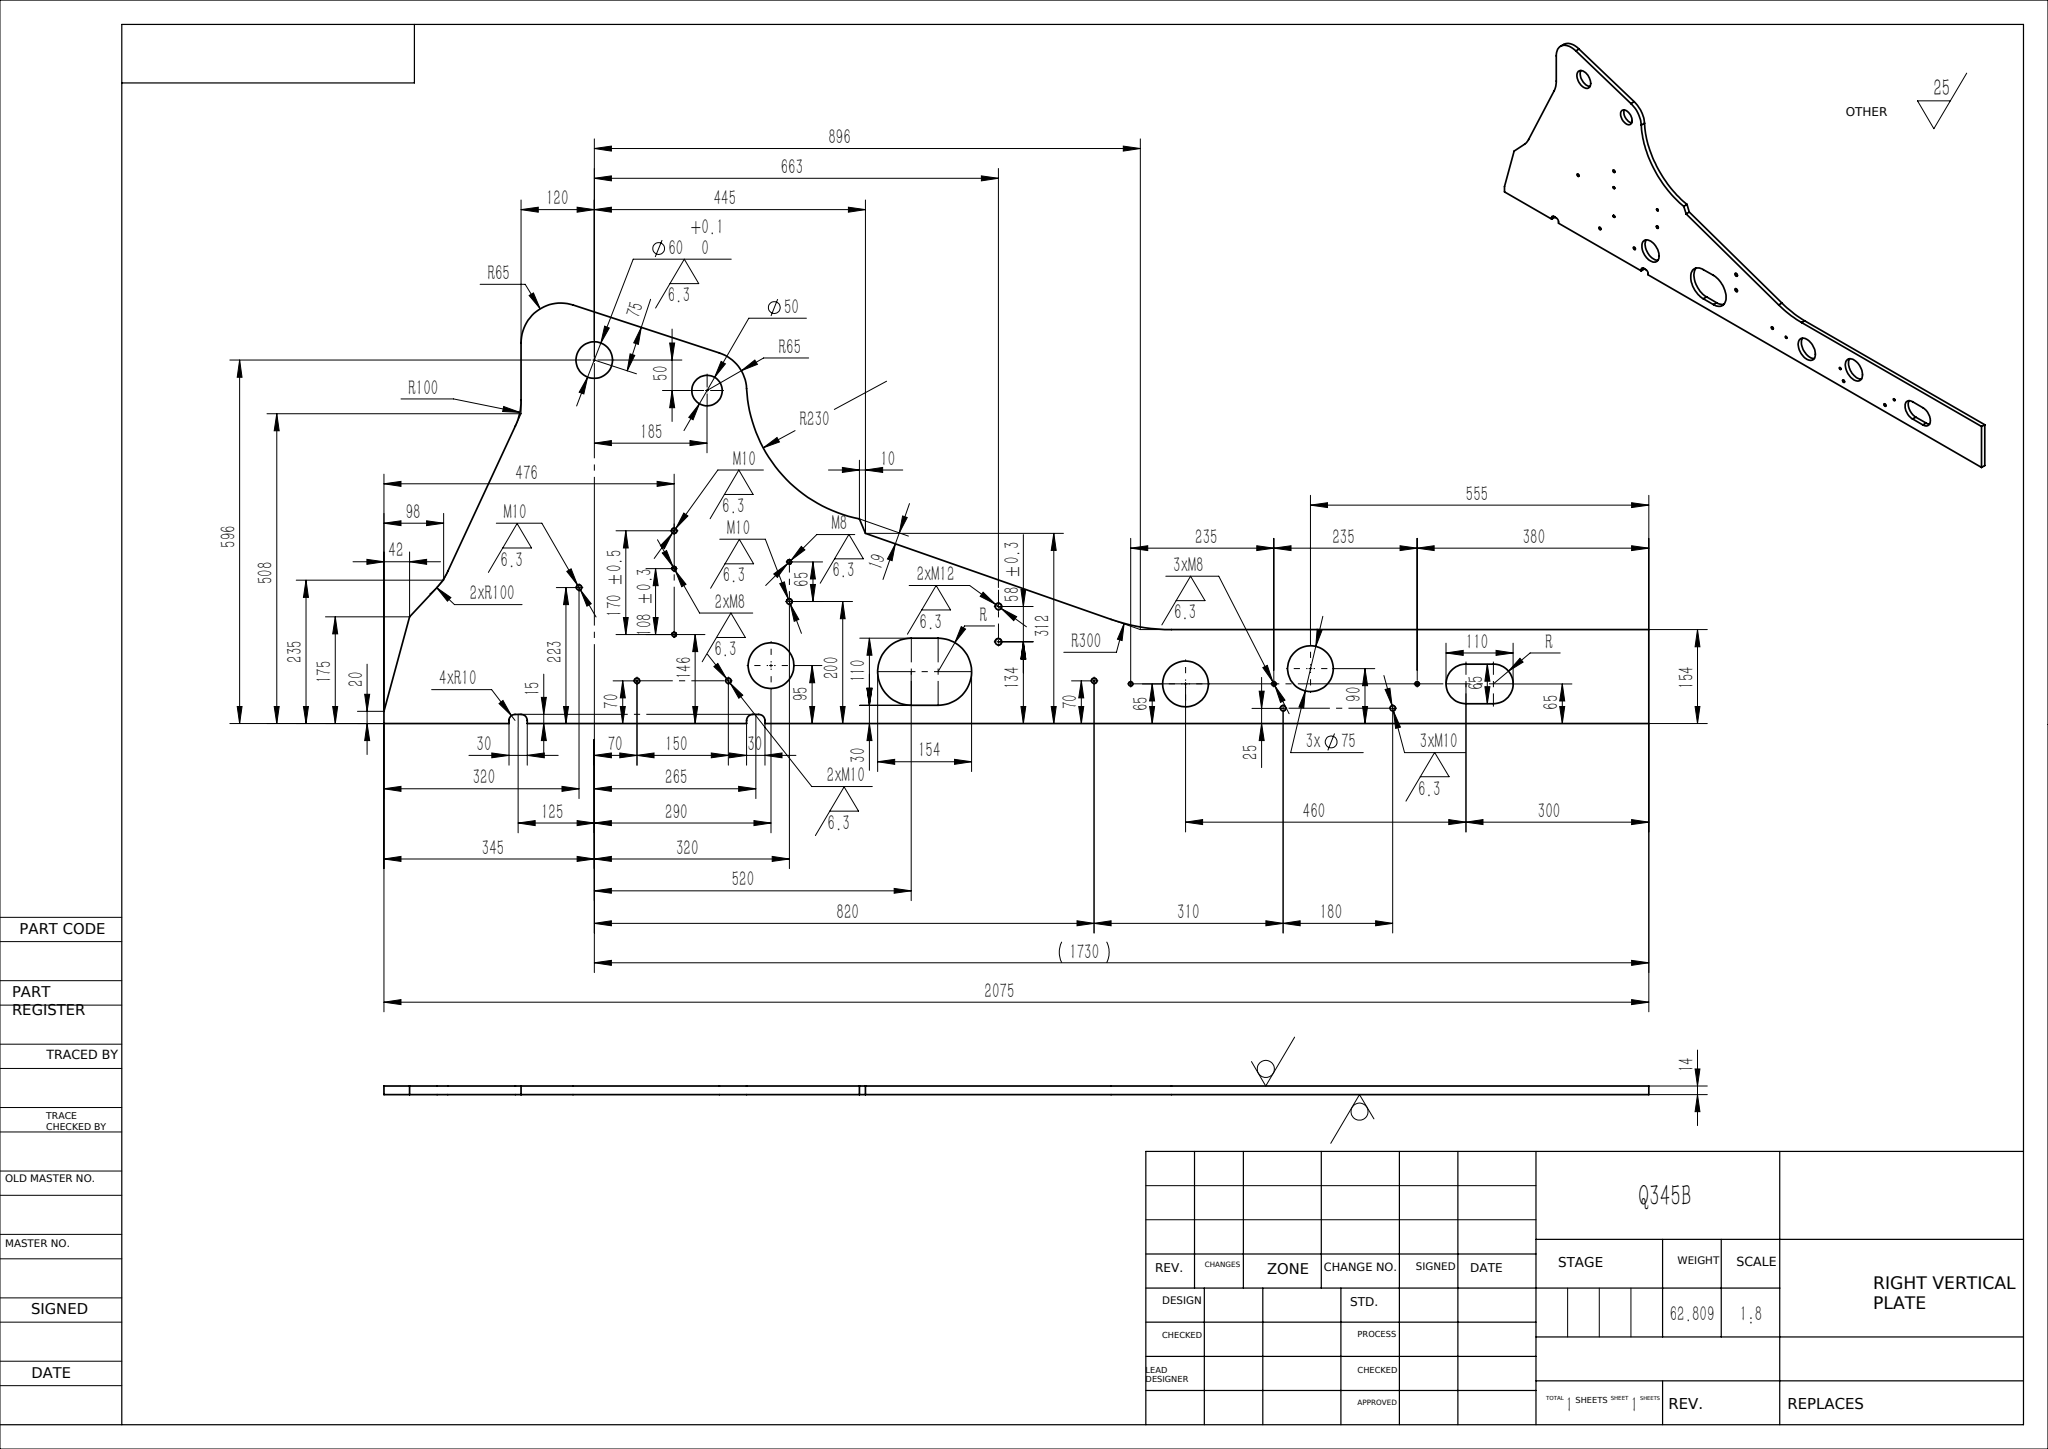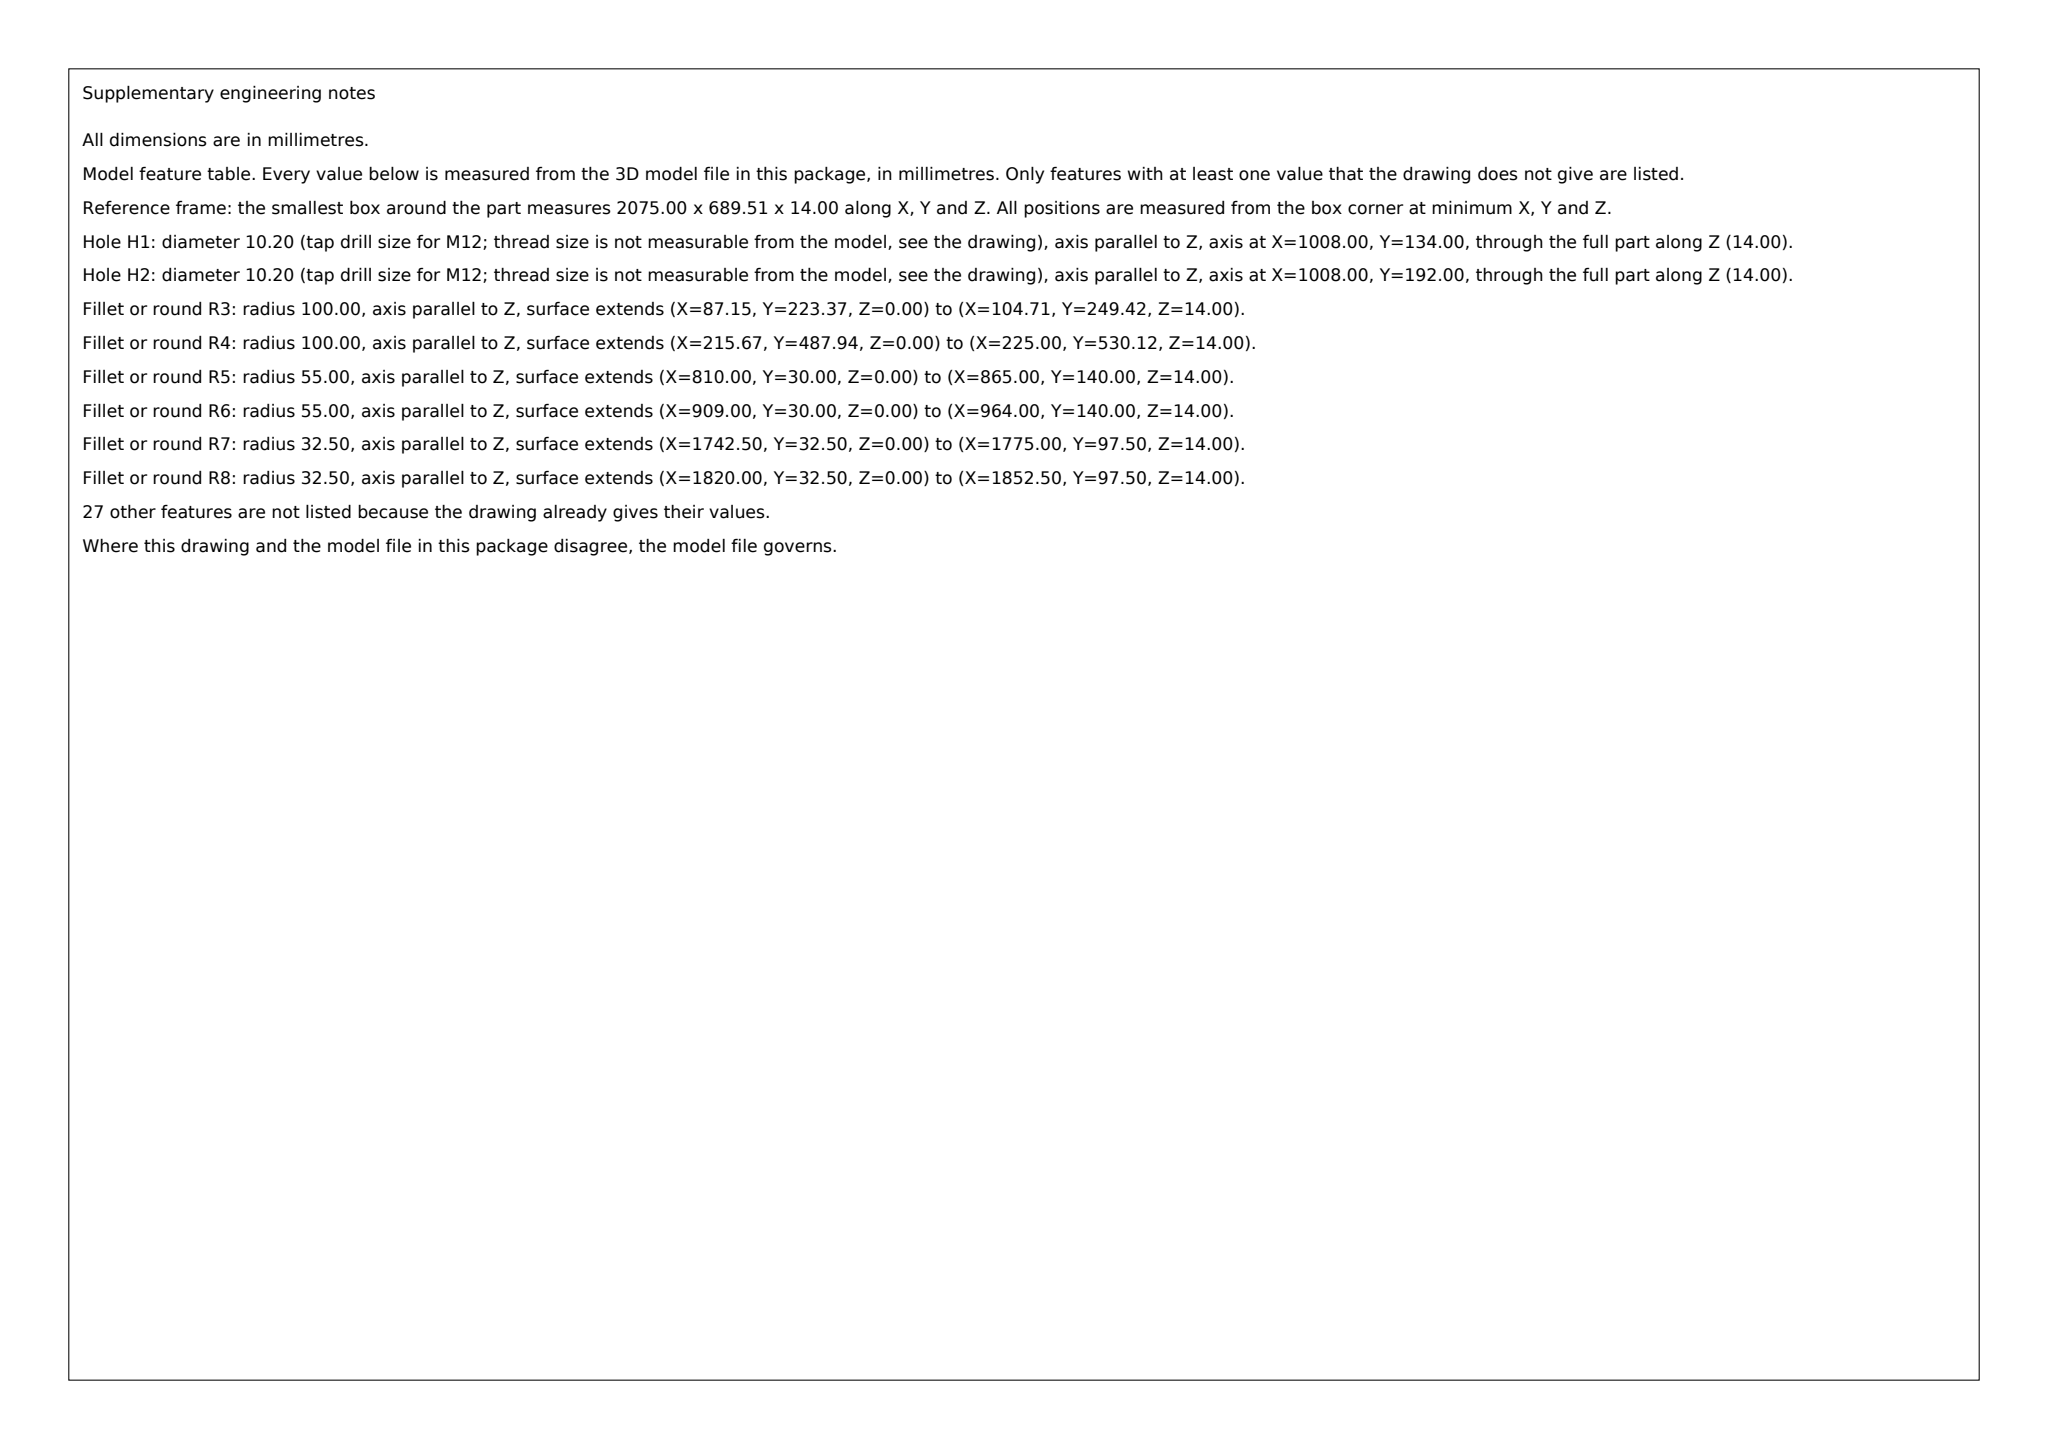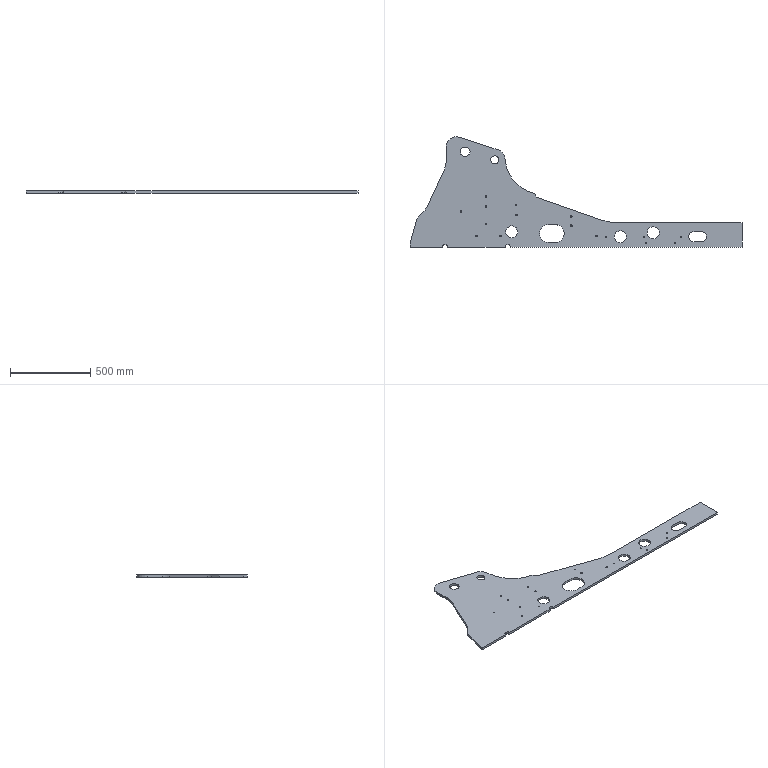Part | SolidWorks | mm | material Q345B | 1 solid | 83 faces | box 2075 x 689.51 x 14 mm | volume 8001084 mm3 | cylinder 58 | plane 25 | commonest cylinder face diameters 8.5 x16 6.8 x12 75 x6 10.2 x4 20 x4 110 x3 65 x3 50 x2
build123d program:
from build123d import *

# Parameters (mm, degrees)
SKETCH1_R           = 30
SKETCH1_R_2         = 37.5
SKETCH1_R_3         = 25
BOSS_EXTRUDE1_DEPTH = 14
M10_TAPPED_HOLE1_D  = 8.5
M10_TAPPED_HOLE2_D  = 8.5
M8_TAPPED_HOLE1_D   = 6.8
M10_TAPPED_HOLE4_D  = 8.5
M8_TAPPED_HOLE3_D   = 6.8
M12_TAPPED_HOLE1_D  = 10.2
M10_TAPPED_HOLE3_D  = 8.5
M8_TAPPED_HOLE4_D   = 6.8


with BuildPart() as part:
    # Sketch1 → Boss-Extrude1 (new body)
    with BuildSketch(Plane.XY):
        with BuildLine():
            Line((0, 0), (205, 0))
            Line((205, 0), (205, 5))
            ThreePointArc((205, 5), (207.929, 12.071), (215, 15))
            Line((215, 15), (225, 15))
            ThreePointArc((225, 15), (232.071, 12.071), (235, 5))
            Line((235, 5), (235, 0))
            Line((235, 0), (595, 0))
            Line((595, 0), (595, 5))
            ThreePointArc((595, 5), (597.929, 12.071), (605, 15))
            Line((605, 15), (615, 15))
            ThreePointArc((615, 15), (622.071, 12.071), (625, 5))
            Line((625, 5), (625, 0))
            Line((625, 0), (2075, 0))
            Line((2075, 0), (2075, 154))
            Line((2075, 154), (1292.029, 154))
            ThreePointArc((1292.029, 154), (1241.723, 158.248), (1192.84, 170.872))
            Line((1192.84, 170.872), (790, 312))
            Line((790, 312), (780, 335.636))
            ThreePointArc((780, 335.636), (650.738, 410.702), (594.913, 549.364))
            ThreePointArc((594.913, 549.364), (581.619, 585.503), (550.21, 607.778))
            Line((550.21, 607.778), (310.21, 686.293))
            ThreePointArc((310.21, 686.293), (251.847, 677.139), (225, 624.514))
            Line((225, 624.514), (225, 530.122))
            ThreePointArc((225, 530.122), (222.639, 508.522), (215.669, 487.942))
            Line((215.669, 487.942), (104.71, 249.423))
            ThreePointArc((104.71, 249.423), (96.957, 235.703), (87.146, 223.371))
            Line((87.146, 223.371), (42, 175))
            Line((42, 175), (0, 20))
            Line((0, 20), (0, 0))
        make_face()
        with Locations((345, 596)):
            Circle(SKETCH1_R, mode=Mode.SUBTRACT)
        with Locations((1520, 90)):
            Circle(SKETCH1_R_2, mode=Mode.SUBTRACT)
        with Locations((1315, 65)):
            Circle(SKETCH1_R_2, mode=Mode.SUBTRACT)
        with Locations((635, 95)):
            Circle(SKETCH1_R_2, mode=Mode.SUBTRACT)
        with Locations((530, 546)):
            Circle(SKETCH1_R_3, mode=Mode.SUBTRACT)
        with BuildLine():
            Line((1775, 97.5), (1820, 97.5))
            ThreePointArc((1820, 97.5), (1852.5, 65), (1820, 32.5))
            Line((1820, 32.5), (1775, 32.5))
            ThreePointArc((1775, 32.5), (1742.5, 65), (1775, 97.5))
        make_face(mode=Mode.SUBTRACT)
        with BuildLine():
            Line((865, 140), (909, 140))
            ThreePointArc((909, 140), (964, 85), (909, 30))
            Line((909, 30), (865, 30))
            ThreePointArc((865, 30), (810, 85), (865, 140))
        make_face(mode=Mode.SUBTRACT)
    extrude(amount=BOSS_EXTRUDE1_DEPTH)

    # M10 Tapped Hole1 (through all)
    with Locations(Plane(origin=(320, 223, 14), x_dir=(1, 0, 0), z_dir=(0, 0, 1))):
        with Locations((0, 0), (95, -153), (245, -153)):
            Hole(M10_TAPPED_HOLE1_D / 2)

    # M10 Tapped Hole2 (through all)
    with Locations(Plane(origin=(476, 316, 14), x_dir=(1, 0, 0), z_dir=(0, 0, 1))):
        with Locations((0, 0)):
            Hole(M10_TAPPED_HOLE2_D / 2)

    # M8 Tapped Hole1 (through all)
    with Locations(Plane(origin=(476, 254, 14), x_dir=(1, 0, 0), z_dir=(0, 0, 1))):
        with Locations((0, 0), (189, 11)):
            Hole(M8_TAPPED_HOLE1_D / 2)

    # M10 Tapped Hole4 (through all)
    with Locations(Plane(origin=(665, 200, 14), x_dir=(1, 0, 0), z_dir=(0, 0, 1))):
        with Locations((0, 0)):
            Hole(M10_TAPPED_HOLE4_D / 2)

    # M8 Tapped Hole3 (through all)
    with Locations(Plane(origin=(476, 146, 14), x_dir=(1, 0, 0), z_dir=(0, 0, 1))):
        with Locations((0, 0)):
            Hole(M8_TAPPED_HOLE3_D / 2)

    # M12 Tapped Hole1 (through all)
    with Locations(Plane(origin=(1008, 192, 14), x_dir=(1, 0, 0), z_dir=(0, 0, 1))):
        with Locations((0, 0), (0, -58)):
            Hole(M12_TAPPED_HOLE1_D / 2)

    # M10 Tapped Hole3 (through all)
    with Locations(Plane(origin=(1165, 70, 14), x_dir=(1, 0, 0), z_dir=(0, 0, 1))):
        with Locations((0, 0), (310, -45), (490, -45)):
            Hole(M10_TAPPED_HOLE3_D / 2)

    # M8 Tapped Hole4 (through all)
    with Locations(Plane(origin=(1225, 65, 14), x_dir=(1, 0, 0), z_dir=(0, 0, 1))):
        with Locations((0, 0), (235, 0), (470, 0)):
            Hole(M8_TAPPED_HOLE4_D / 2)


solid = part.part